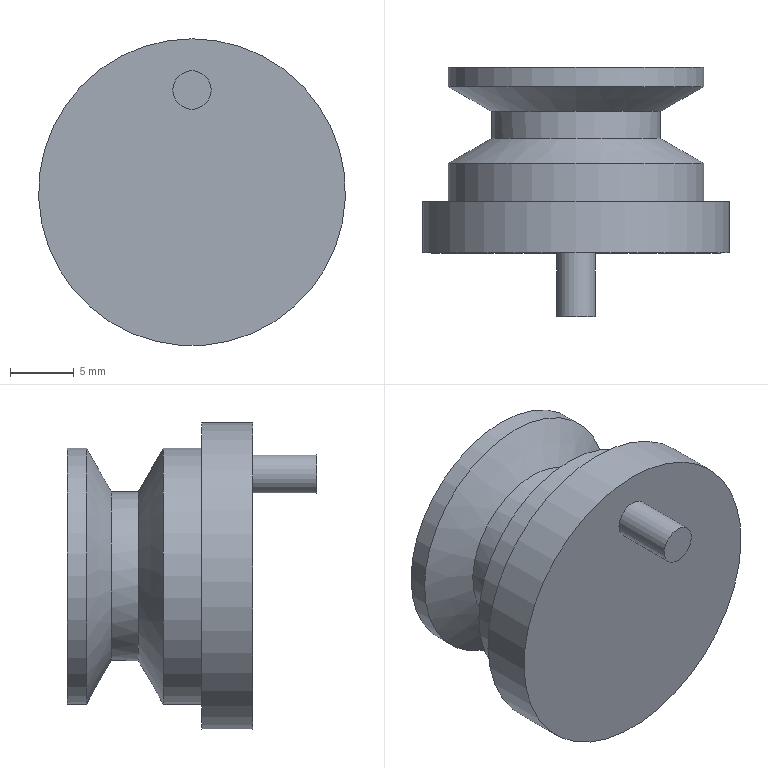Component | NX | MODEL3 | 1 solid | 18 faces | volume 3519 mm3 | cylinder 7 | plane 6 | spline 3 | cone 2 | commonest cylinder face diameters 20 x2 13.235 x1 24 x1 3 x1 8.5 x1 10 x1